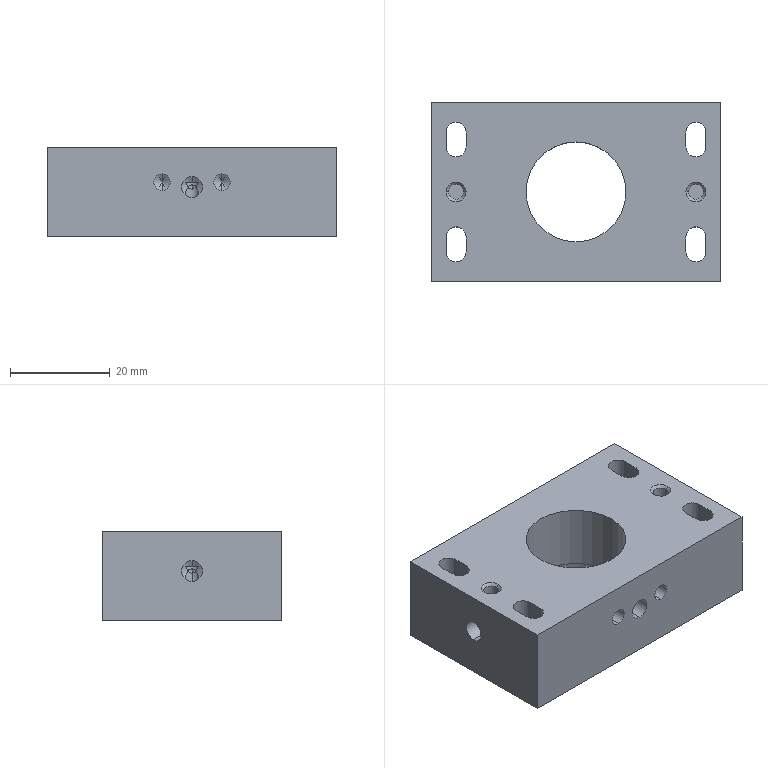Component | SolidWorks | SpacerBlock-1 | 1 solid | 86 faces | box 58 x 36 x 18 mm | volume 27082 mm3 | cylinder 45 | plane 21 | cone 20 | commonest cylinder face diameters 3 x17 3.3 x8 4.2 x8 4 x8 30 x2 20 x2
build123d program:
from build123d import *

# Parameters (mm, degrees)
SKETCH1_W                  = 58
SKETCH1_H                  = 36
EXTRUDE1_DEPTH             = 18
CUT_EXTRUDE1_DEPTH         = 39.588
SKETCH4_R                  = 1.5
EXTRUDE2_DEPTH             = 4
CHAMFER1_SIZE              = 0.5
SKETCH5_R                  = 10
EXTRUDE3_DEPTH             = 39.588
SKETCH6_R                  = 15
EXTRUDE5_DEPTH             = 5
M4_TAPPED_HOLE1_AT_2_COUNT = 2
M4_TAPPED_HOLE1_AT_2_PITCH = 12
SKETCH12_R                 = 1.5
EXTRUDE6_DEPTH             = 6
CIRCULAR_PATTERN1_COUNT    = 4


with BuildPart() as part:
    # Sketch1 → Extrude1 (new body)
    with BuildSketch(Plane.XY):
        Rectangle(SKETCH1_W, SKETCH1_H)
    extrude(amount=EXTRUDE1_DEPTH)

    # Sketch3 → Cut-Extrude1 (cut, through all)
    with BuildSketch(Plane.XY.offset(18)):
        with BuildLine():
            Line((22, 12), (22, 9))
            ThreePointArc((22, 9), (24, 7), (26, 9))
            Line((26, 9), (26, 12))
            ThreePointArc((26, 12), (24, 14), (22, 12))
        make_face()
        with BuildLine():
            Line((22, -9), (22, -12))
            ThreePointArc((22, -12), (24, -14), (26, -12))
            Line((26, -12), (26, -9))
            ThreePointArc((26, -9), (24, -7), (22, -9))
        make_face()
        with BuildLine():
            Line((-22, -12), (-22, -9))
            ThreePointArc((-22, -9), (-24, -7), (-26, -9))
            Line((-26, -9), (-26, -12))
            ThreePointArc((-26, -12), (-24, -14), (-22, -12))
        make_face()
        with BuildLine():
            Line((-22, 9), (-22, 12))
            ThreePointArc((-22, 12), (-24, 14), (-26, 12))
            Line((-26, 12), (-26, 9))
            ThreePointArc((-26, 9), (-24, 7), (-22, 9))
        make_face()
    extrude(amount=-CUT_EXTRUDE1_DEPTH, mode=Mode.SUBTRACT)

    # Sketch4 → Extrude2 (cut)
    with BuildSketch(Plane.XY.offset(18)):
        with Locations((-24, 0)):
            Circle(SKETCH4_R)
        with Locations((24, 0)):
            Circle(SKETCH4_R)
    extrude(amount=-EXTRUDE2_DEPTH, mode=Mode.SUBTRACT)

    # Chamfer1
    chamfer1_edges = [part.edges().sort_by_distance(p)[0] for p in [
        (-25.5, 0, 18),
        (22.5, 0, 18),
    ]]
    chamfer(chamfer1_edges, length=CHAMFER1_SIZE)

    # Sketch5 → Extrude3 (cut, through all)
    with BuildSketch(Plane.XY.offset(18)):
        Circle(SKETCH5_R)
    extrude(amount=-EXTRUDE3_DEPTH, mode=Mode.SUBTRACT)

    # Sketch6 → Extrude5 (cut)
    with BuildSketch(Plane(origin=(0, 0, 0), x_dir=(-1, 0, 0), z_dir=(0, 0, -1))):
        Circle(SKETCH6_R)
    extrude(amount=-EXTRUDE5_DEPTH, mode=Mode.SUBTRACT)

    # Sketch7 → M4 Tapped Hole1 (revolve, cut)
    with BuildSketch(Plane(origin=(-6, 18, 11), x_dir=(0, 0, 1), z_dir=(1, 0, 0))):
        Polygon((0, 0), (0, 9.491), (1.65, 8.5), (1.65, 0), align=None)
    m4_tapped_hole1 = revolve(axis=Axis((-6, 24.35, 11), (0, -1, 0)), mode=Mode.SUBTRACT)

    # M4 Tapped Hole1 at 2: M4 Tapped Hole1 ×2
    with Locations(*[(i * M4_TAPPED_HOLE1_AT_2_PITCH, 0, 0) for i in range(1, M4_TAPPED_HOLE1_AT_2_COUNT)]):
        add(m4_tapped_hole1, mode=Mode.SUBTRACT)

    # Sketch10 → M5 Tapped Hole1 (revolve, cut)
    with BuildSketch(Plane(origin=(-29, 0, 10), x_dir=(0, 0, 1), z_dir=(0, 1, 0))):
        Polygon((0, 0), (0, 18.262), (2.1, 17), (2.1, 0), align=None)
    m5_tapped_hole1 = revolve(axis=Axis((-35.35, 0, 10), (1, 0, 0)), mode=Mode.SUBTRACT)

    # Sketch12 → Extrude6 (cut)
    with BuildSketch(Plane(origin=(0, 0, 5), x_dir=(-1, 0, 0), z_dir=(0, 0, -1))):
        with Locations((12.5, 0)):
            Circle(SKETCH12_R)
    extrude6 = extrude(amount=-EXTRUDE6_DEPTH, mode=Mode.SUBTRACT)

    # Circular Pattern1: Extrude6 ×4 about axis
    circular_pattern1_axis = Axis((0, 0, 0), (0, 0, 1))
    for i in range(1, CIRCULAR_PATTERN1_COUNT):
        add(extrude6.rotate(circular_pattern1_axis, i * 360 / CIRCULAR_PATTERN1_COUNT), mode=Mode.SUBTRACT)

    # Sketch13 → M5 Tapped Hole2 (revolve, cut)
    with BuildSketch(Plane(origin=(0, 18, 10), x_dir=(0, 0, 1), z_dir=(1, 0, 0))):
        Polygon((0, 0), (0, 7.262), (2.1, 6), (2.1, 0), align=None)
    m5_tapped_hole2 = revolve(axis=Axis((0, 24.35, 10), (0, -1, 0)), mode=Mode.SUBTRACT)

    # Mirror1: M5 Tapped Hole2 across plane
    add(m5_tapped_hole2.mirror(Plane.ZX), mode=Mode.SUBTRACT)

    # Mirror2: M5 Tapped Hole1 across plane
    add(m5_tapped_hole1.mirror(Plane(origin=(0, 0, 0), x_dir=(0, 0, 1), z_dir=(1, 0, 0))), mode=Mode.SUBTRACT)

    # Mirror3: M4 Tapped Hole1 across plane
    add(m4_tapped_hole1.mirror(Plane.ZX), mode=Mode.SUBTRACT)

    # Mirror3 copy 1 sketch → Mirror3 copy 1 (revolve, cut)
    with BuildSketch(Plane(origin=(6, -18, 11), x_dir=(0, 0, 1), z_dir=(1, 0, 0))):
        Polygon((0, 0), (0, -9.491), (1.65, -8.5), (1.65, 0), align=None)
    revolve(axis=Axis((6, -24.35, 11), (0, -1, 0)), mode=Mode.SUBTRACT)


solid = part.part

# Placed as in the assembly
solid = solid.moved(Location((-50, 135.5, -164.197), (0, 0, 0)))